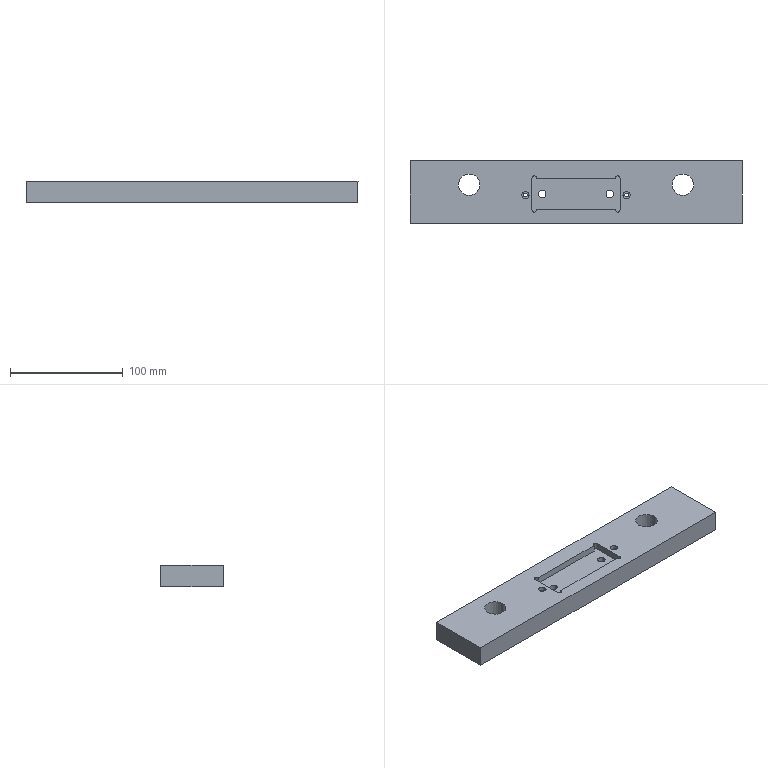Component | SolidWorks | 2SZT-2-006-3 | 1 solid | 47 faces | box 295 x 55.5 x 19.01 mm | volume 283700 mm3 | cylinder 30 | plane 17 | commonest cylinder face diameters 4 x6 11 x4 6.5 x4 3.4 x4 10 x4 19.02 x4 6.6 x4
build123d program:
from build123d import *

# Parameters (mm, degrees)
SKETCH1_W                                            = 55.5
SKETCH1_H                                            = 19
BOSS_EXTRUDE1_DEPTH                                  = 295
SKETCH5_R                                            = 9.51
CUT_EXTRUDE2_DEPTH                                   = 301.776
SKETCH6_R                                            = 5
CUT_EXTRUDE3_DEPTH                                   = 7
F_1_0_1_DIAMETER_HOLE1_D                             = 1
F_1_0_1_DIAMETER_HOLE1_DEPTH                         = 20
F_1_0_1_DIAMETER_HOLE1_TIP                           = 0.3004
M3_HEX_SOCKET_HEAD_CAP_SCREW_CBORE1_D                = 3.4
M3_HEX_SOCKET_HEAD_CAP_SCREW_CBORE1_CBORE_D          = 6.5
M3_HEX_SOCKET_HEAD_CAP_SCREW_CBORE1_CBORE_DEPTH      = 3.4
HOLE_SIZE_ACCORDING_TO_THE_TYPE_OF_HEXAG_D           = 6.6
HOLE_SIZE_ACCORDING_TO_THE_TYPE_OF_HEXAG_CBORE_D     = 11
HOLE_SIZE_ACCORDING_TO_THE_TYPE_OF_HEXAG_CBORE_DEPTH = 6.8
SKETCH19_W                                           = 28.2
SKETCH19_H                                           = 78.2
CUT_EXTRUDE4_DEPTH                                   = 6
SKETCH20_R                                           = 2
CUT_EXTRUDE5_DEPTH                                   = 6


with BuildPart() as part:
    # Sketch1 → Boss-Extrude1 (new body)
    with BuildSketch(Plane.XY):
        with Locations((27.75, -9.5)):
            Rectangle(SKETCH1_W, SKETCH1_H)
    extrude(amount=BOSS_EXTRUDE1_DEPTH)

    # Sketch5 → Cut-Extrude2 (cut, through all)
    with BuildSketch(Plane(origin=(0, 0, 0), x_dir=(1, 0, 0), z_dir=(0, 1, 0))):
        with Locations(Location((34.192, -52.5, 0), (0, 0, 270))):
            Circle(SKETCH5_R)
        with Locations(Location((34.192, -242.5, 0), (0, 0, 270))):
            Circle(SKETCH5_R)
    extrude(amount=-CUT_EXTRUDE2_DEPTH, mode=Mode.SUBTRACT)

    # Sketch6 → Cut-Extrude3 (cut)
    with BuildSketch(Plane(origin=(0, 0, 0), x_dir=(1, 0, 0), z_dir=(0, 1, 0))):
        with Locations(Location((25, -102.5, 0), (0, 0, 270))):
            Circle(SKETCH6_R)
        with Locations(Location((25, -192.5, 0), (0, 0, 270))):
            Circle(SKETCH6_R)
    extrude(amount=-CUT_EXTRUDE3_DEPTH, mode=Mode.SUBTRACT)

    # 1.0 _1_ Diameter Hole1
    with Locations(Plane(origin=(0, -7, 0), x_dir=(1, 0, 0), z_dir=(0, 1, 0))):
        with Locations((25, -102.5), (25, -192.5)):
            Hole(F_1_0_1_DIAMETER_HOLE1_D / 2, depth=F_1_0_1_DIAMETER_HOLE1_DEPTH)
            with Locations((0, 0, -(F_1_0_1_DIAMETER_HOLE1_DEPTH + F_1_0_1_DIAMETER_HOLE1_TIP / 2))):  # 118° drill point
                Cone(0, F_1_0_1_DIAMETER_HOLE1_D / 2, F_1_0_1_DIAMETER_HOLE1_TIP, mode=Mode.SUBTRACT)

    # M3 Hex Socket Head Cap Screw CBORE1 (through all)
    with Locations(Plane(origin=(0, -19, 0), x_dir=(-1, 0, 0), z_dir=(0, -1, 0))):
        with Locations((-25, -192.5), (-25, -102.5)):
            CounterBoreHole(M3_HEX_SOCKET_HEAD_CAP_SCREW_CBORE1_D / 2, M3_HEX_SOCKET_HEAD_CAP_SCREW_CBORE1_CBORE_D / 2, M3_HEX_SOCKET_HEAD_CAP_SCREW_CBORE1_CBORE_DEPTH)

    # Hole Size according to the type of hexag (through all)
    with Locations(Plane(origin=(0, 0, 0), x_dir=(1, 0, 0), z_dir=(0, 1, 0))):
        with Locations((25.95, -177.5), (25.95, -117.5)):
            CounterBoreHole(HOLE_SIZE_ACCORDING_TO_THE_TYPE_OF_HEXAG_D / 2, HOLE_SIZE_ACCORDING_TO_THE_TYPE_OF_HEXAG_CBORE_D / 2, HOLE_SIZE_ACCORDING_TO_THE_TYPE_OF_HEXAG_CBORE_DEPTH)

    # Sketch19 → Cut-Extrude4 (cut)
    with BuildSketch(Plane(origin=(0, -19, 0), x_dir=(-1, 0, 0), z_dir=(0, -1, 0))):
        with Locations((-25.95, -147.5)):
            Rectangle(SKETCH19_W, SKETCH19_H)
    extrude(amount=-CUT_EXTRUDE4_DEPTH, mode=Mode.SUBTRACT)

    # Sketch20 → Cut-Extrude5 (cut)
    with BuildSketch(Plane.XZ.offset(19)):
        with Locations((11.85, 184.6)):
            Circle(SKETCH20_R)
        with Locations((40.05, 184.6)):
            Circle(SKETCH20_R)
        with Locations((40.05, 110.4)):
            Circle(SKETCH20_R)
        with Locations((11.85, 110.4)):
            Circle(SKETCH20_R)
    extrude(amount=-CUT_EXTRUDE5_DEPTH, mode=Mode.SUBTRACT)


solid = part.part

# Placed as in the assembly
solid = solid.moved(Location((1102.766, 350.193, -293.265), (-90, -90, 0)))